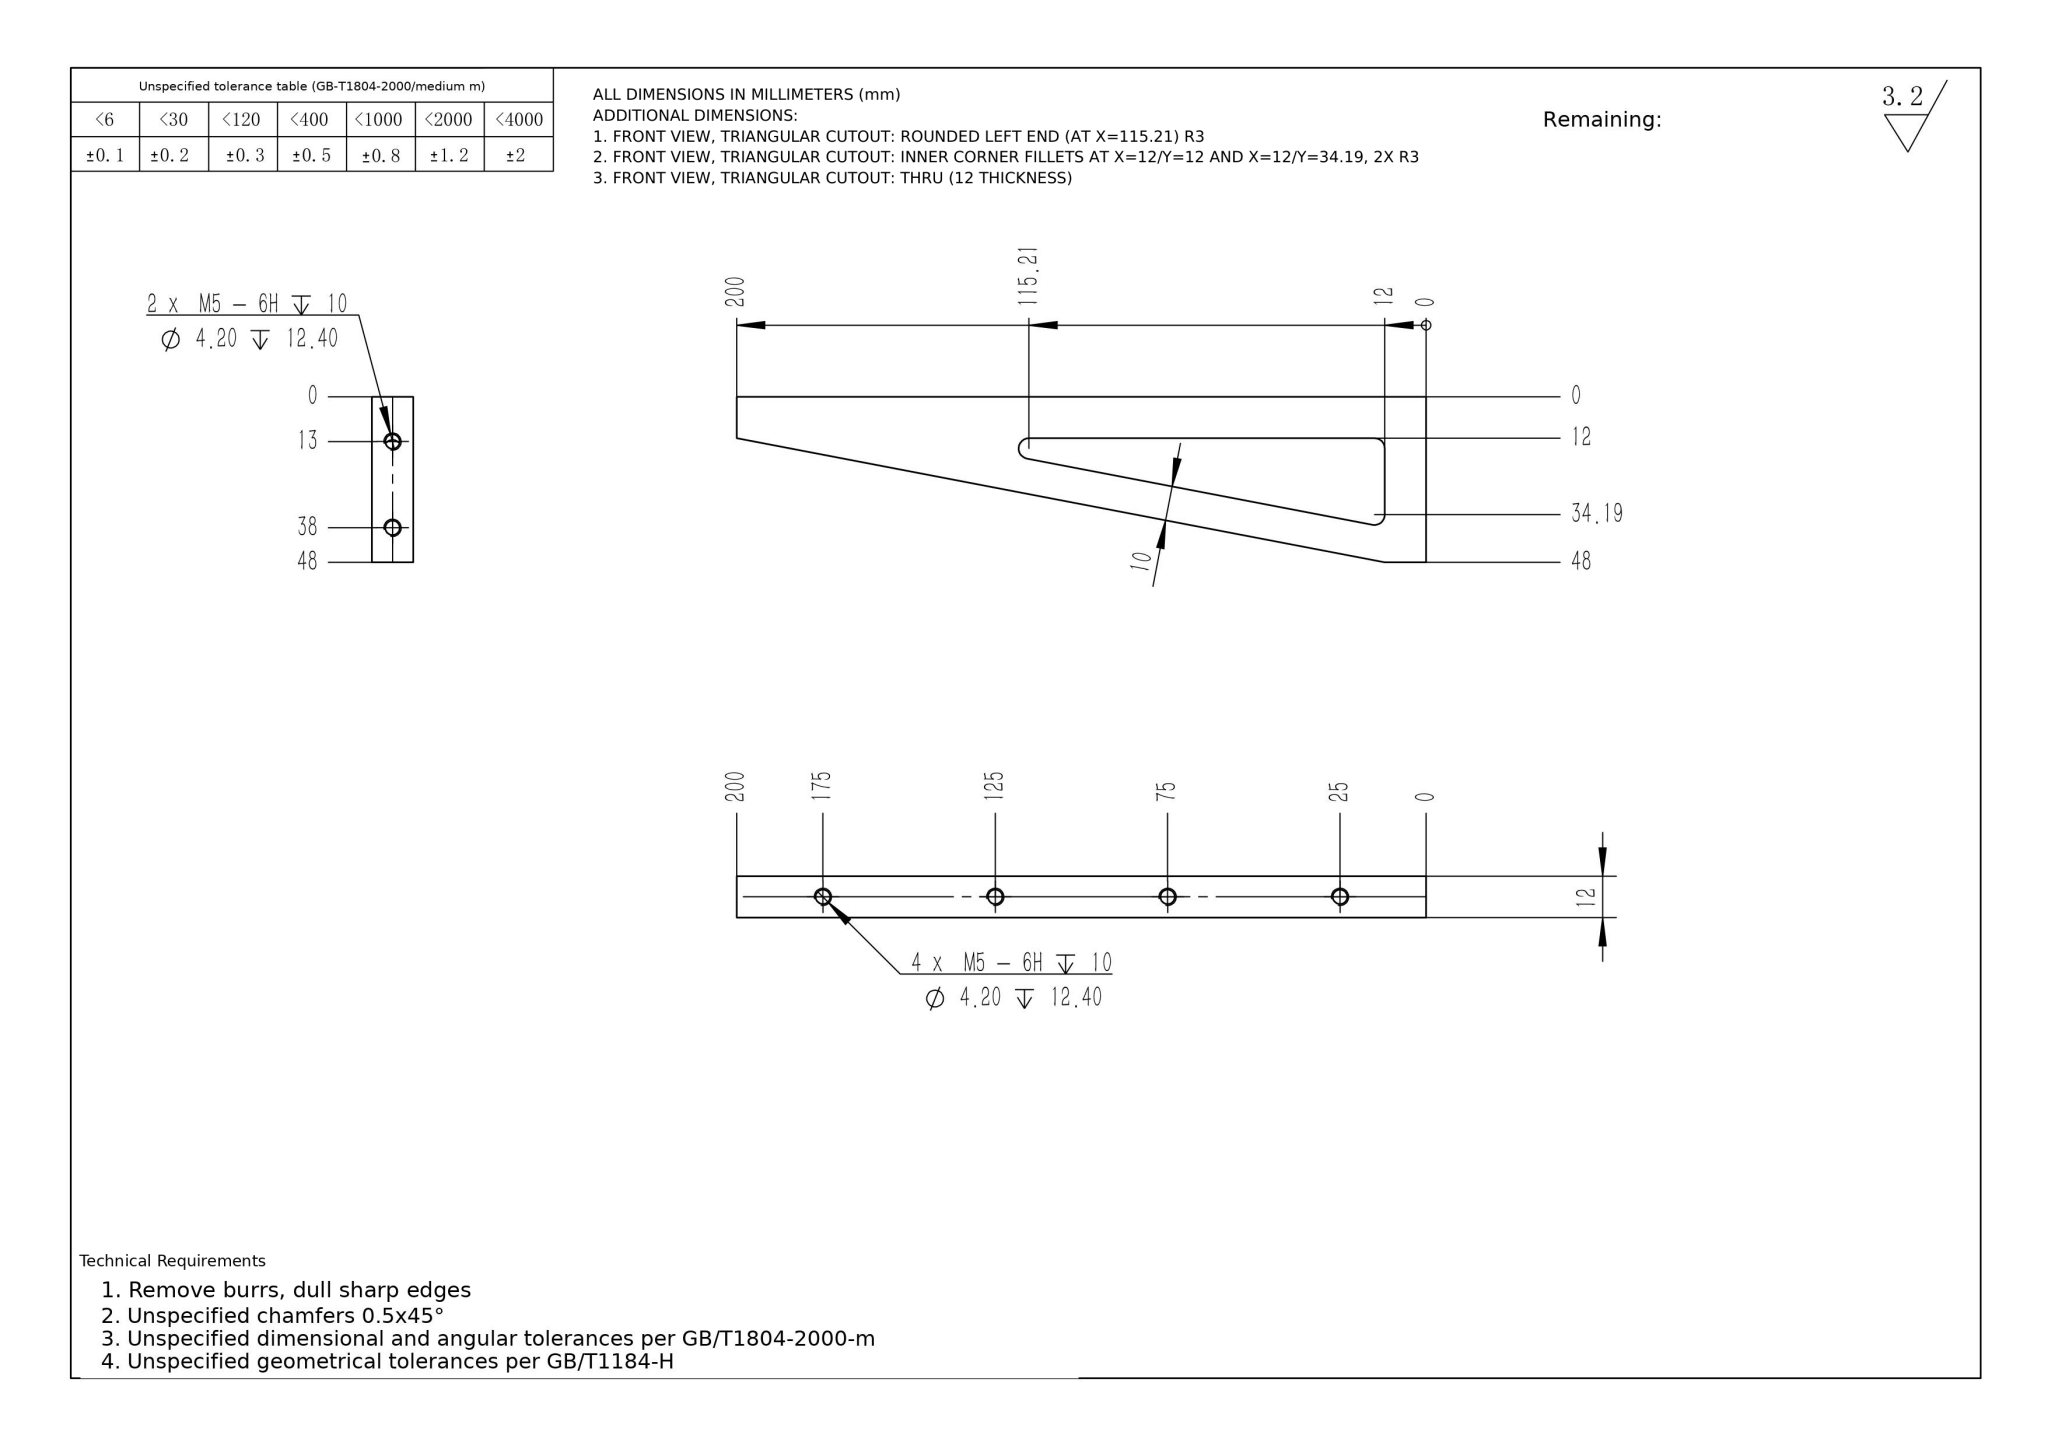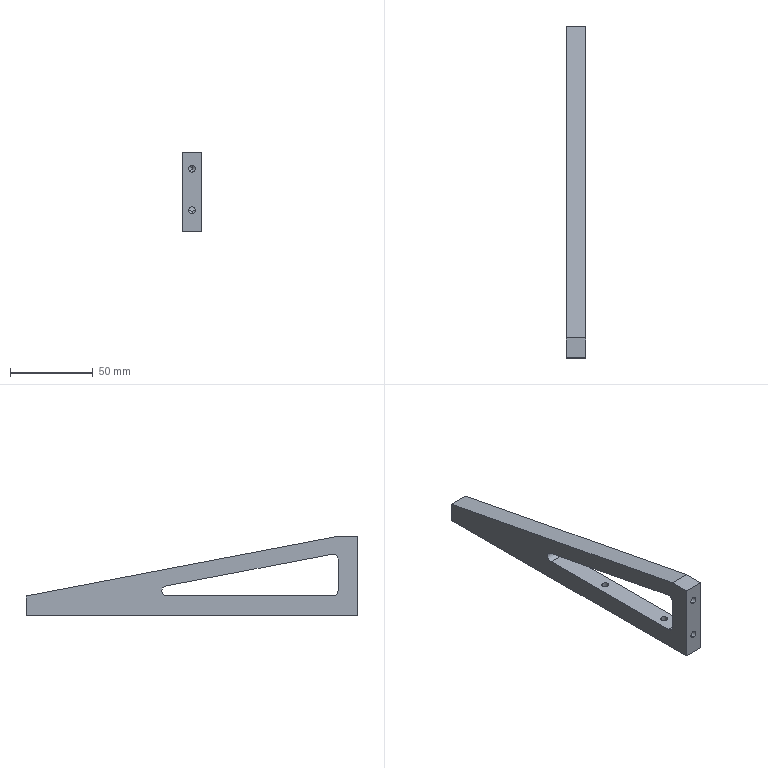Part | NX | mm | 1 solid | 34 faces | box 12 x 200 x 48 mm | volume 53704 mm3 | cylinder 16 | plane 10 | cone 8 | commonest cylinder face diameters 4.2 x12 6 x4